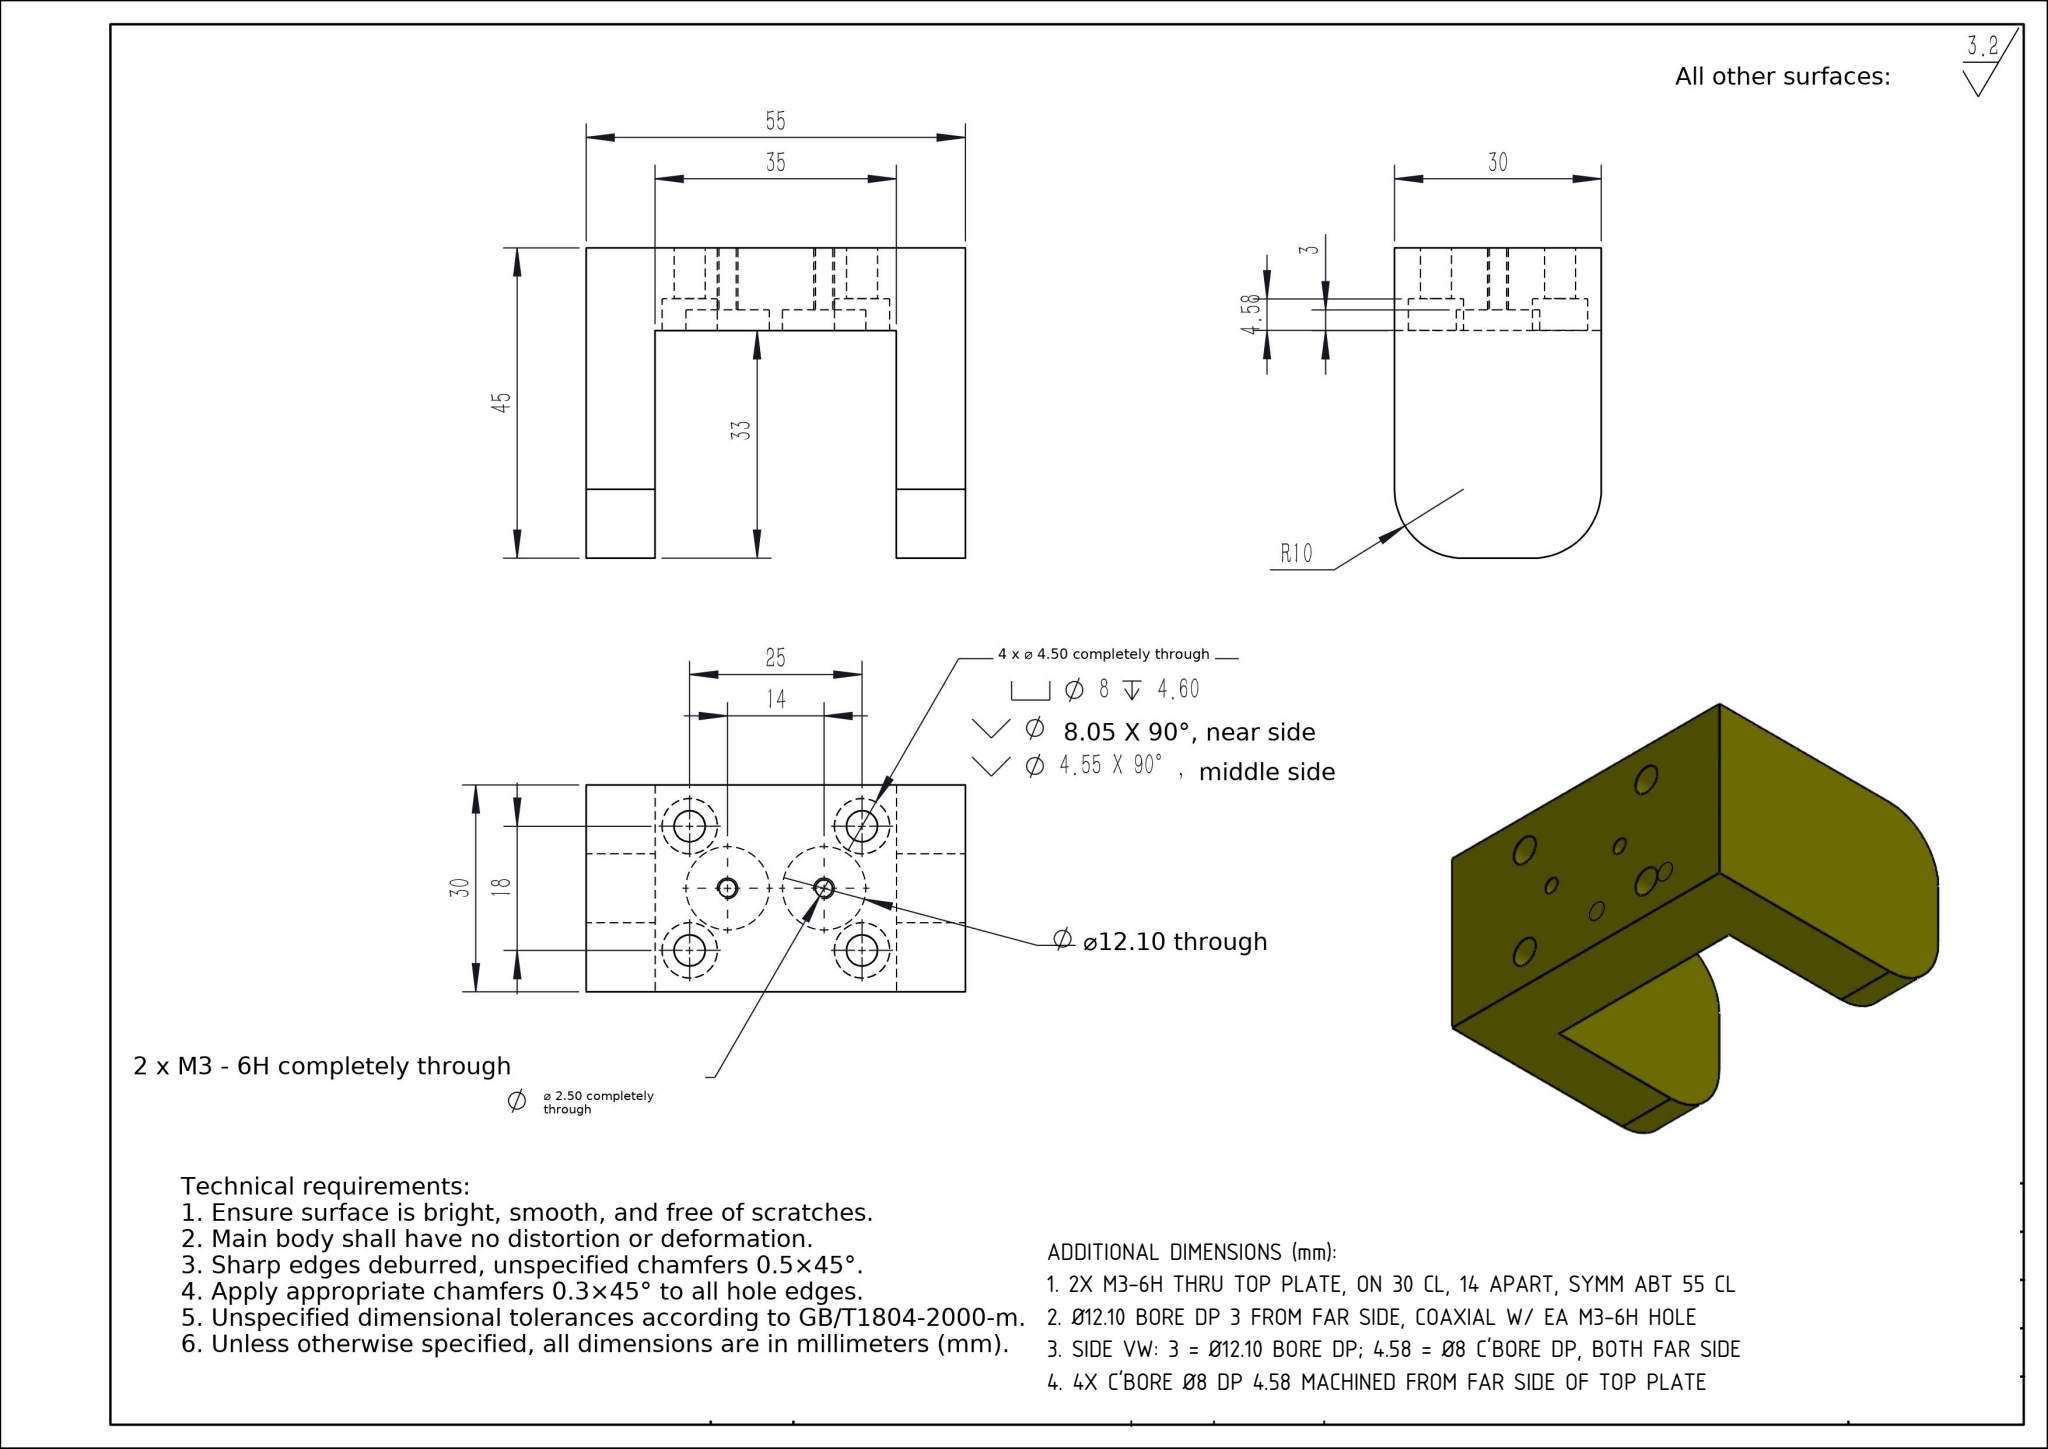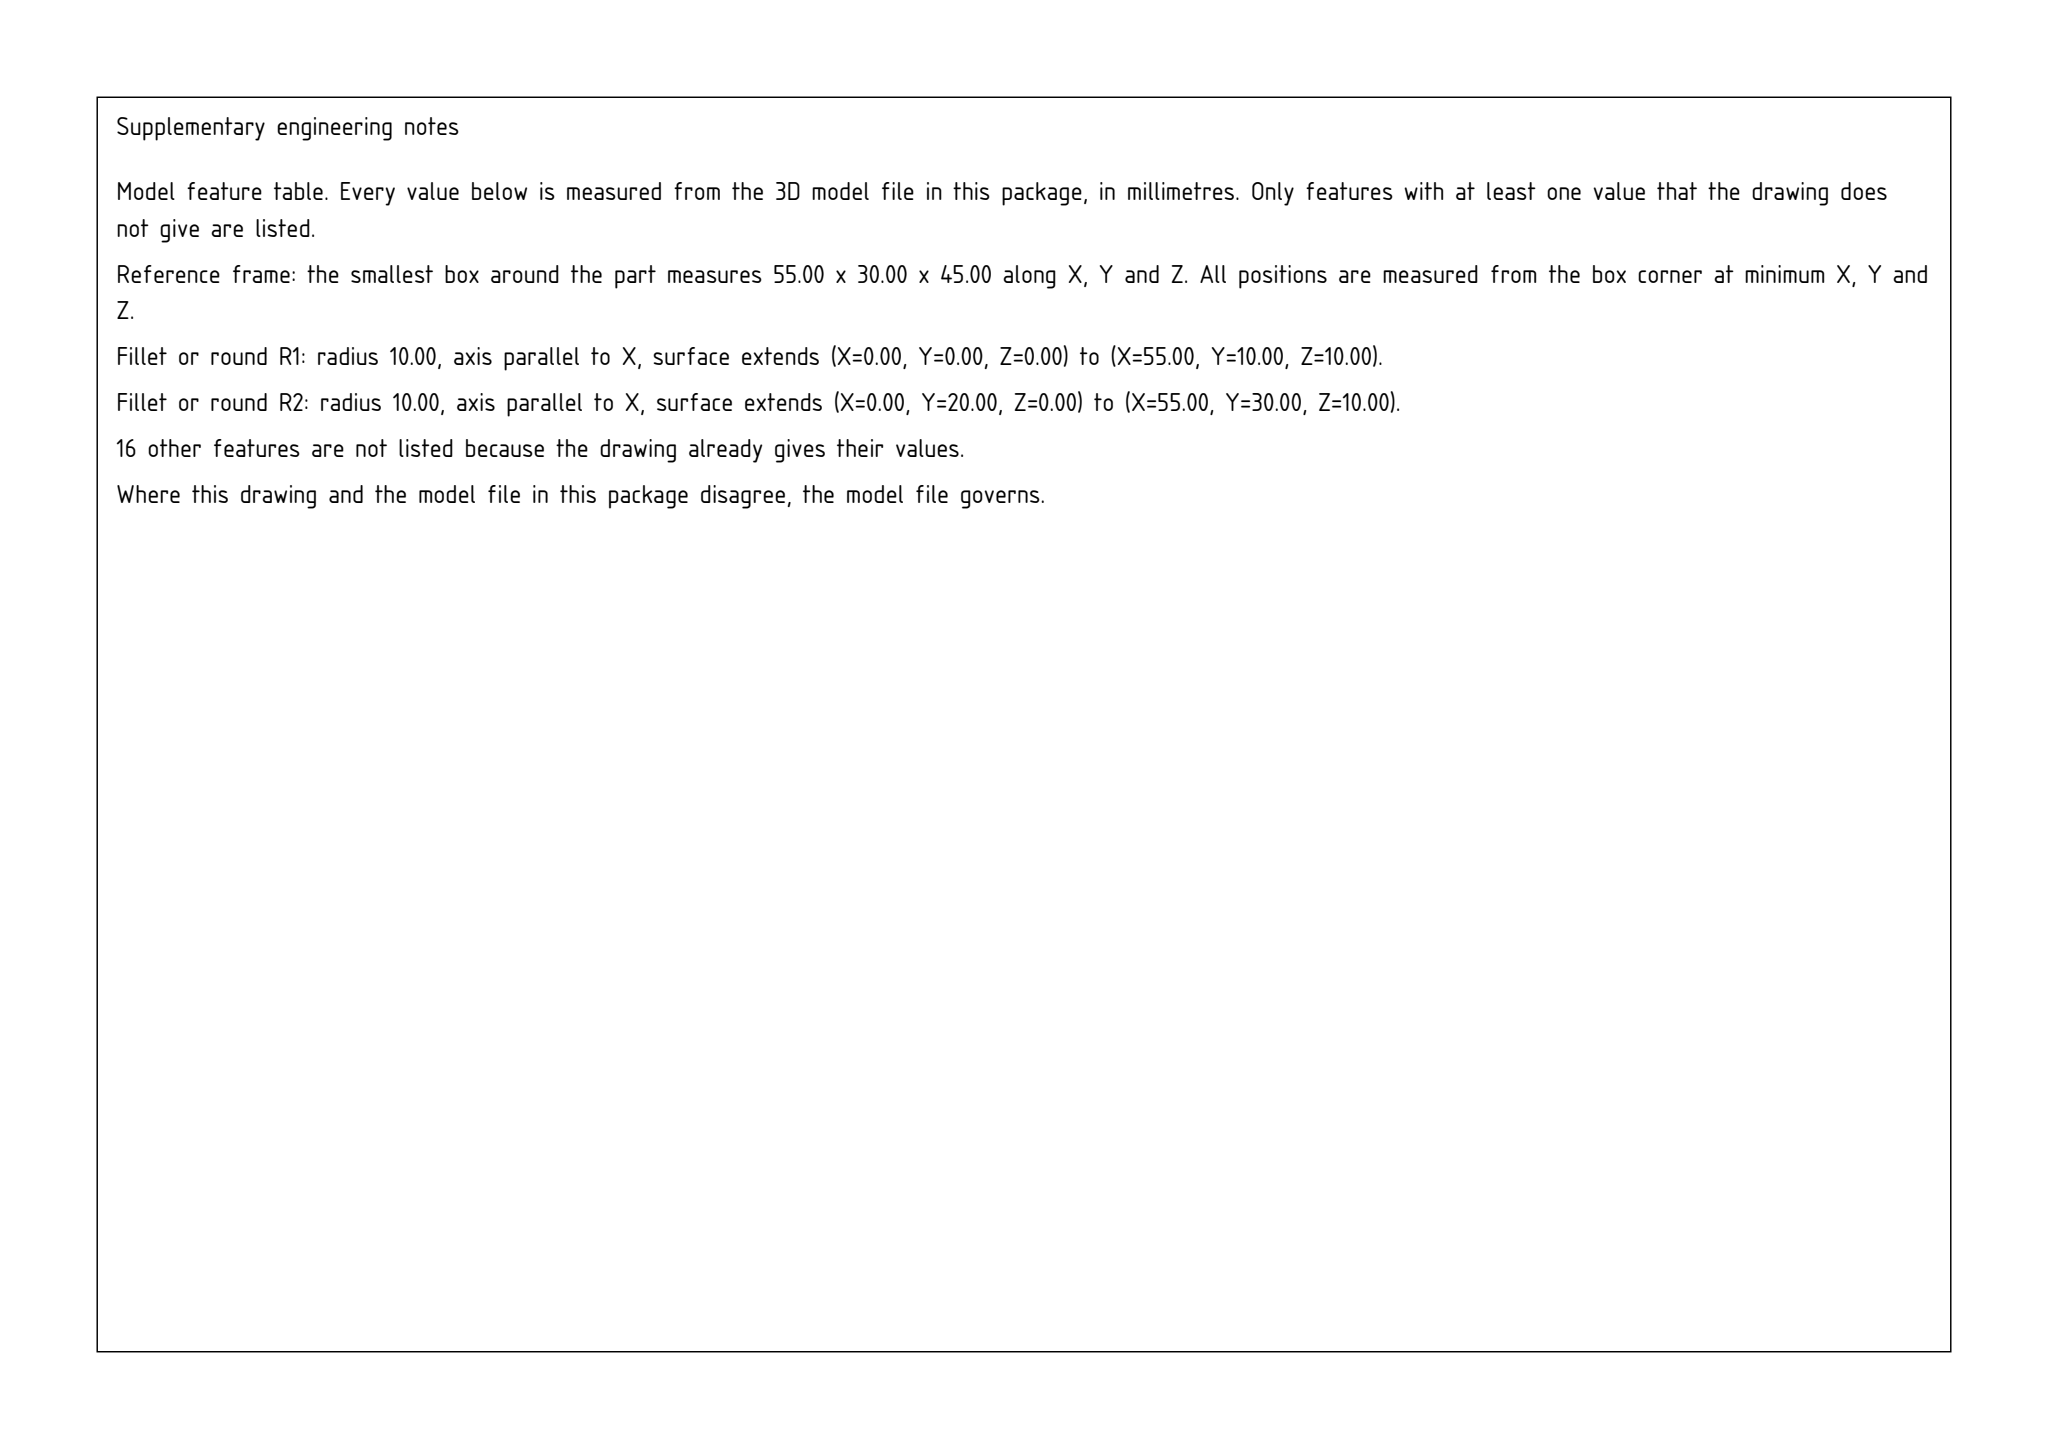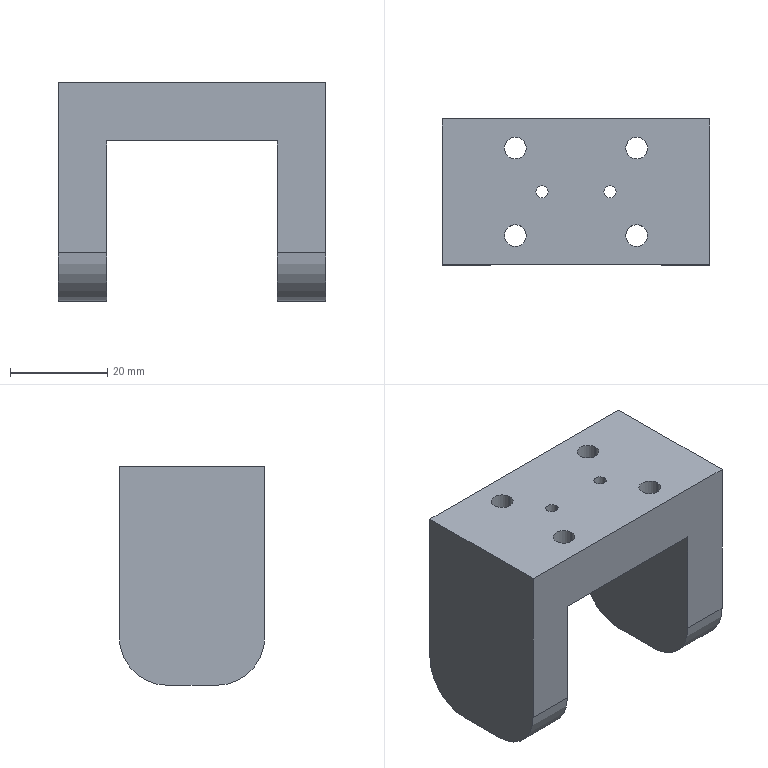Part | SolidWorks | mm | 1 solid | 60 faces | box 55 x 30 x 45 mm | volume 36568 mm3 | cylinder 28 | cone 16 | plane 16 | commonest cylinder face diameters 8 x8 4.5 x8 2.5 x4 12.1 x4 20 x4
build123d program:
from build123d import *

# Parameters (mm, degrees)
EXTRUDE_THIN1_DEPTH                       = 30
FILLET1_R                                 = 10
MOVE_FACE1_BY                             = 2
HOLE_SIZE_ACCORDING_TO_HEXAGON_SO_2_COUNT = 2
HOLE_SIZE_ACCORDING_TO_HEXAGON_SO_2_PITCH = 25
HOLE_SIZE_ACCORDING_TO_HEXAGON_SO_3_COUNT = 2
HOLE_SIZE_ACCORDING_TO_HEXAGON_SO_3_PITCH = 30.806
HOLE_SIZE_ACCORDING_TO_HEXAGON_SO_4_COUNT = 2
HOLE_SIZE_ACCORDING_TO_HEXAGON_SO_4_PITCH = 18
SKETCH4_R                                 = 6.05
CUT_EXTRUDE1_DEPTH                        = 3
M3_TAPPED_HOLE1_D                         = 2.5


with BuildPart() as part:
    # Sketch1 → Extrude-Thin1 (new body)
    with BuildSketch(Plane(origin=(0, 0, 0), x_dir=(1, 0, 0), z_dir=(0, 1, 0))):
        Polygon((0, 35), (0, 0), (35, 0), (35, 35), (45, 35), (45, -10), (-10, -10), (-10, 35), align=None)
    extrude(amount=EXTRUDE_THIN1_DEPTH)

    # Fillet1
    fillet1_edges = [part.edges().sort_by_distance(p)[0] for p in [
        (-5, 30, -35),
        (40, 30, -35),
        (-5, 0, -35),
        (40, 0, -35),
    ]]
    fillet(fillet1_edges, radius=FILLET1_R)

    # Move Face1: a face moved outward by 2.0
    extrude(part.faces().sort_by_distance((17.5, 15, 0))[0], amount=MOVE_FACE1_BY, dir=(0, 0, -1))

    # Sketch2 → Hole Size _ according to_ Hexagon Socket (revolve, cut)
    with BuildSketch(Plane(origin=(30, 24, -2), x_dir=(0, 1, 0), z_dir=(1, 0, 0))):
        Polygon((0, 0), (0, 12), (2.25, 12), (2.25, 4.625), (2.275, 4.6), (4, 4.6), (4, 0.025), (4.025, 0), align=None)
    hole_size_according_to_hexagon_socket = revolve(axis=Axis((30, 24, -8.35), (0, 0, 1)), mode=Mode.SUBTRACT)

    # Hole Size _ according to_ Hexagon So 2: Hole Size _ according to_ Hexagon Socket ×2
    with Locations(*[(-i * HOLE_SIZE_ACCORDING_TO_HEXAGON_SO_2_PITCH, 0, 0) for i in range(1, HOLE_SIZE_ACCORDING_TO_HEXAGON_SO_2_COUNT)]):
        add(hole_size_according_to_hexagon_socket, mode=Mode.SUBTRACT)

    # Hole Size _ according to_ Hexagon So 3: Hole Size _ according to_ Hexagon Socket ×2
    with Locations(*[Vector(-0.8115, -0.5843, 0) * (i * HOLE_SIZE_ACCORDING_TO_HEXAGON_SO_3_PITCH) for i in range(1, HOLE_SIZE_ACCORDING_TO_HEXAGON_SO_3_COUNT)]):
        add(hole_size_according_to_hexagon_socket, mode=Mode.SUBTRACT)

    # Hole Size _ according to_ Hexagon So 4: Hole Size _ according to_ Hexagon Socket ×2
    with Locations(*[(0, -i * HOLE_SIZE_ACCORDING_TO_HEXAGON_SO_4_PITCH, 0) for i in range(1, HOLE_SIZE_ACCORDING_TO_HEXAGON_SO_4_COUNT)]):
        add(hole_size_according_to_hexagon_socket, mode=Mode.SUBTRACT)

    # Sketch4 → Cut-Extrude1 (cut)
    with BuildSketch(Plane(origin=(0, 0, -2), x_dir=(-1, 0, 0), z_dir=(0, 0, -1))):
        with Locations((-24.5, 15)):
            Circle(SKETCH4_R)
        with Locations((-10.5, 15)):
            Circle(SKETCH4_R)
    extrude(amount=-CUT_EXTRUDE1_DEPTH, mode=Mode.SUBTRACT)

    # M3 Tapped Hole1 (through all)
    with Locations(Plane(origin=(0, 0, 1), x_dir=(-1, 0, 0), z_dir=(0, 0, -1))):
        with Locations((-24.5, 15), (-10.5, 15)):
            Hole(M3_TAPPED_HOLE1_D / 2)


solid = part.part